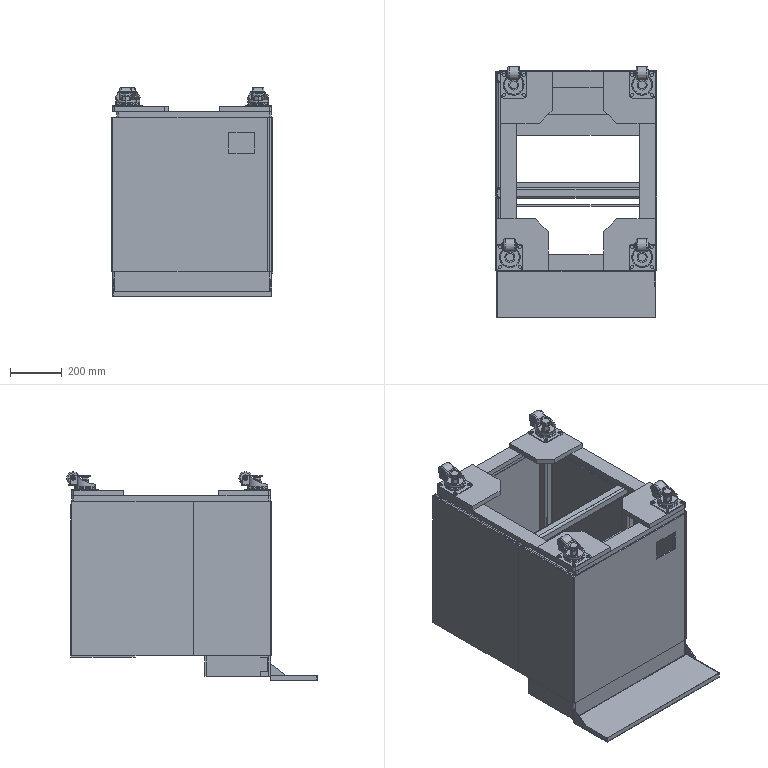Assembly | SolidWorks | mm | 31 component files | 63 solids | 1320 faces | box 625 x 971.67 x 809 mm | volume 27248260 mm3 | plane 703 | cylinder 457 | cone 96 | torus 64 | commonest cylinder face diameters 16 x106 8 x80 11 x48 13 x32 20 x20 80 x16 24 x16 25 x16
Bill of materials:
CMAS50_Fadjuster | 4 | 45 | Headed pin or bolt-like part: a thin, wide, round head with a slightly tapered underside, a hexagonal neck section under the head, and a long plain cylindrical shank with a chamfered end.
CMAS50_Fbearing | 4 | 45 | Stepped cylinder: a large main cylinder with a shorter, smaller coaxial cylindrical spigot sticking out of each end.
CMAS50_Fbody | 4 | 45 | Bracket with a circular base and a central hexagonal boss with a through-hole. A curved wall rises from the base to two parallel upright ears, each with a round boss or pivot feature.
CMAS50_Fswivel | 4 | 45 | Square flange plate with rounded corners, four slotted holes at the corners, and a raised circular disc with a central round through-hole.
CMAS50_Fwheel | 4 | 45 | Cylindrical sleeve or bushing with a central through-bore and rounded outer edges.
CoverPlate1 | 2 |  | Thin flat rectangular plate, about twice as long as it is wide, with no visible features.
CoverPlate2 | 2 |  | Thin flat rectangular plate, slightly taller than it is wide, with no visible features.
CoverPlate3 | 1 |  | Thin flat square plate with one small rectangular through-cutout near one corner.
CoverPlate4 | 1 |  | Thin flat square plate with no visible features.
CoverPlate5 | 1 |  | Thin flat rectangular strip or panel, about 3.5 times as long as it is wide, with no visible features.
CoverPlate6 | 2 |  | Long, narrow, thin flat strip or bar with no visible features.
ItemTray | 1 |  | Rectangular plate with a thin triangular flange or gusset standing up at each short end, placed toward one long edge.
STRack | 1 |  | Open rectangular box frame made of square/rectangular bar members: four vertical corner posts, top and bottom perimeter rails, and an intermediate vertical post with a cross rail that splits the frame into two bays. Square corner plates with chamfered inner corners and a single small hole each sit on the top corners. A flat vertical panel with a few small holes fills part of one side, and a solid rectangular base block sits under one corner.
Mates:
1. coincident | STRack-1 face at (-277, 602, 620) dir (0, 0, 1) | CMAS50_F-4/CMAS50_Fswivel-1 face at (-273, 520, 620) dir (0, 0, -1)
2. coincident | STRack-1 face at (-285, 602, 620) dir (-1, 0, 0) | CMAS50_F-4/CMAS50_Fswivel-1 face at (-285, 520, 623.2) dir (-1, 0, 0)
3. coincident | STRack-1 face at (-277, 610, 620) dir (0, 1, 0) | CMAS50_F-4/CMAS50_Fswivel-1 face at (-273, 610, 623.2) dir (0, 1, 0)
4. coincident | STRack-1 face at (307, 602, 620) dir (0, 0, 1) | CMAS50_F-2/CMAS50_Fswivel-1 face at (225, 520, 620) dir (0, 0, -1)
5. coincident | STRack-1 face at (315, 602, 620) dir (1, 0, 0) | CMAS50_F-2/CMAS50_Fswivel-1 face at (315, 598, 623.2) dir (1, 0, 0)
6. coincident | STRack-1 face at (307, 610, 620) dir (0, 1, 0) | CMAS50_F-2/CMAS50_Fswivel-1 face at (225, 610, 623.2) dir (0, 1, 0)
7. coincident | STRack-1 face at (-292, -152, 620) dir (0, 0, 1) | CMAS50_F-3/CMAS50_Fswivel-1 face at (-288, -148, 620) dir (0, 0, -1)
8. coincident | STRack-1 face at (-300, -152, 620) dir (-1, 0, 0) | CMAS50_F-3/CMAS50_Fswivel-1 face at (-300, -148, 623.2) dir (-1, 0, 0)
9. coincident | STRack-1 face at (-292, -160, 620) dir (0, -1, 0) | CMAS50_F-3/CMAS50_Fswivel-1 face at (-210, -160, 623.2) dir (0, -1, 0)
10. coincident | STRack-1 face at (-300, 140, 12) dir (-1, 0, 0) | CoverPlate1-1 face at (-300, -10, 280) dir (1, 0, 0)
11. coincident | STRack-1 edge at (-285, 602, 580) dir (0, -1, 0) | CoverPlate1-1 face at (-300, -160, 580) dir (0, 0, 1)
12. coincident | STRack-1 face at (-292, -160, 560) dir (0, -1, 0) | CoverPlate1-1 face at (-300, -160, 580) dir (0, -1, 0)
13. coincident | STRack-1 face at (315, 152, 560) dir (1, 0, 0) | CoverPlate1-2 face at (315, -10, 280) dir (-1, 0, 0)
14. coincident | STRack-1 face at (0, 0, 580) dir (0, 0, -1) | CoverPlate1-2 face at (320, -160, 580) dir (0, 0, 1)
15. coincident | STRack-1 face at (283, -160, 560) dir (0, -1, 0) | CoverPlate1-2 face at (320, -160, 580) dir (0, -1, 0)
16. coincident | STRack-1 face at (315, 590, 548) dir (1, 0, 0) | CoverPlate2-1 face at (315, 375, 280) dir (-1, 0, 0)
17. coincident | CoverPlate1-2 face at (320, 140, 580) dir (0, 1, 0) | CoverPlate2-1 face at (320, 140, 580) dir (0, -1, 0)
18. coincident | STRack-1 face at (283, 180, -20) dir (0, 0, -1) | CoverPlate2-1 face at (320, 140, -20) dir (0, 0, -1)
19. coincident | STRack-1 face at (-300, 180, -12) dir (-1, 0, 0) | CoverPlate2-2 face at (-300, 375, 280) dir (1, 0, 0)
20. coincident | CoverPlate1-1 face at (-300, 140, 580) dir (0, 1, 0) | CoverPlate2-2 face at (-300, 140, 580) dir (0, -1, 0)
21. coincident | STRack-1 face at (0, 0, 580) dir (0, 0, -1) | CoverPlate2-2 face at (-300, 140, 580) dir (0, 0, 1)
22. coincident | STRack-1 face at (-280, -160, 548) dir (0, -1, 0) | CoverPlate3-1 face at (0, -160, 280) dir (0, 1, 0)
23. coincident | STRack-1 face at (0, 0, 580) dir (0, 0, -1) | CoverPlate3-1 face at (-300, -160, 580) dir (0, 0, 1)
24. coincident | CoverPlate1-1 face at (-300, -10, 280) dir (1, 0, 0) | CoverPlate3-1 face at (-300, -160, -20) dir (-1, 0, 0)
25. coincident | STRack-1 face at (295, 610, 548) dir (0, 1, 0) | CoverPlate4-1 face at (15, 610, 272.5) dir (0, -1, 0)
26. tangent | STRack-1 face at (295, 578, -12) dir (-1, 0, 0) r 8 | CoverPlate4-1 face at (-285, 615, -20) dir (0, 0, -1)
27. coincident | CoverPlate2-1 face at (315, 375, 280) dir (-1, 0, 0) | CoverPlate4-1 face at (315, 615, -20) dir (1, 0, 0)
28. coincident | STRack-1 face at (-292, 180, -20) dir (0, 0, -1) | CoverPlate5-1 face at (15, 530, -20) dir (0, 0, 1)
29. coincident | CoverPlate2-1 face at (320, 375, 280) dir (1, 0, 0) | CoverPlate5-1 face at (320, 615, -20) dir (1, 0, 0)
30. coincident | CoverPlate4-1 face at (15, 615, 272.5) dir (0, 1, 0) | CoverPlate5-1 face at (-290, 615, -20) dir (0, 1, 0)
31. coincident | STRack-1 face at (0, 90, 0) dir (0, 1, 0) | CoverPlate6-1 face at (15, 90, -60) dir (0, -1, 0)
32. coincident | STRack-1 face at (283, -140, -20) dir (0, 0, -1) | CoverPlate6-1 face at (-285, 95, -20) dir (0, 0, 1)
33. coincident | STRack-1 face at (315, 90, -100) dir (1, 0, 0) | CoverPlate6-1 face at (315, 95, -100) dir (1, 0, 0)
34. coincident | STRack-1 face at (-292, 180, -20) dir (0, 0, -1) | CoverPlate6-2 face at (15, 405, -20) dir (0, 0, 1)
35. coincident | CoverPlate5-1 face at (-290, 445, -20) dir (0, -1, 0) | CoverPlate6-2 face at (-285, 445, -25) dir (0, 1, 0)
36. width | CoverPlate5-1 face at (320, 615, -20) dir (1, 0, 0) | CoverPlate5-1 face at (-290, 615, -20) dir (-1, 0, 0) | CoverPlate6-2 face at (315, 365, -25) dir (1, 0, 0) | CoverPlate6-2 face at (-285, 365, -25) dir (-1, 0, 0)
37. coincident | CMAS50_Fswivel-1 plane at (264, -109, 632.8) dir (0, 0, -1) | CMAS50_Fbody-1 plane at (264, -109, 632.8) dir (0, 0, -1)
38. coincident | CMAS50_Fswivel-1 axis at (264, -109, 570) dir (0, 0, 1) | CMAS50_Fbody-1 axis at (264, -109, 570) dir (0, 0, 1)
39. coincident | CMAS50_Fbody-1 plane at (264, -109, 620) dir (1, 0.009642, 0) | CMAS50_Fbearing-1 plane at (263.556, -63.002, 669) dir (-1, -0.009642, 0)
40. coincident | CMAS50_Fbody-1 axis at (344.453, -62.222, 669) dir (-1, -0.009642, 0) | CMAS50_Fbearing-1 axis at (182.66, -63.782, 669) dir (1, 0.009642, 0)
41. coincident | CMAS50_Fbody-1 axis at (264, -109, 570) dir (0, 0, 1) | CMAS50_Fadjuster-1 axis at (264, -109, 570) dir (0, 0, 1)
42. distance | CMAS50_Fwheel-1 plane at (263.556, -63.002, 669) dir (1, 0.009642, 0) | CMAS50_Fbearing-1 plane at (263.556, -63.002, 669) dir (-1, -0.009642, 0)
43. coincident | CMAS50_Fbearing-1 axis at (182.66, -63.782, 669) dir (1, 0.009642, 0) | CMAS50_Fwheel-1 axis at (344.453, -62.222, 669) dir (-1, -0.009642, 0)
44. coincident | CMAS50_Fbearing-1 axis at (182.66, -63.782, 669) dir (1, 0.009642, 0) | CMAS50_Fwheel-1 axis at (344.453, -62.222, 669) dir (-1, -0.009642, 0)
45. coincident | CMAS50_Fbearing-1 axis at (182.66, -63.782, 669) dir (1, 0.009642, 0) | CMAS50_Fwheel-1 axis at (344.453, -62.222, 669) dir (-1, -0.009642, 0)
46. angle | CMAS50_Fwheel-1 plane at (263.556, -63.002, 669) dir (-0.00848, 0.8794, -0.476) | CMAS50_Fbearing-1 plane at (263.556, -63.002, 669) dir (-0.00848, 0.8794, -0.476)
47. coincident | STRack-1 face at (307, -152, 620) dir (0, 0, 1) | CMAS50_Fswivel-1 face at (225, -148, 620) dir (0, 0, -1)
48. coincident | STRack-1 face at (315, -152, 620) dir (1, 0, 0) | CMAS50_Fswivel-1 face at (315, -70, 623.2) dir (1, 0, 0)
49. coincident | STRack-1 face at (307, -160, 620) dir (0, -1, 0) | CMAS50_Fswivel-1 face at (303, -160, 623.2) dir (0, -1, 0)
50. coincident | CMAS50_Fswivel-1 plane at (0, -12.8, 0) dir (0, 1, 0) | CMAS50_Fbody-1 plane at (0, -12.8, 0) dir (0, 1, 0)
51. coincident | CMAS50_Fswivel-1 axis at (0, 50, 0) dir (0, -1, 0) | CMAS50_Fbody-1 axis at (0, 50, 0) dir (0, -1, 0)
52. coincident | CMAS50_Fbody-1 plane at (0, 0, 0) dir (1, 0, 0.009642) | CMAS50_Fbearing-1 plane at (-0.4435, -49, 45.998) dir (-1, 0, -0.009642)
53. coincident | CMAS50_Fbody-1 axis at (80.453, -49, 46.778) dir (-1, 0, -0.009642) | CMAS50_Fbearing-1 axis at (-81.34, -49, 45.218) dir (1, 0, 0.009642)
54. distance | CMAS50_Fwheel-1 plane at (-0.4435, -49, 45.998) dir (1, 0, 0.009642) | CMAS50_Fbearing-1 plane at (-0.4435, -49, 45.998) dir (-1, 0, -0.009642)
55. coincident | CMAS50_Fbearing-1 axis at (-81.34, -49, 45.218) dir (1, 0, 0.009642) | CMAS50_Fwheel-1 axis at (80.453, -49, 46.778) dir (-1, 0, -0.009642)
56. coincident | CMAS50_Fbearing-1 axis at (-81.34, -49, 45.218) dir (1, 0, 0.009642) | CMAS50_Fwheel-1 axis at (80.453, -49, 46.778) dir (-1, 0, -0.009642)
57. coincident | CMAS50_Fbearing-1 axis at (-81.34, -49, 45.218) dir (1, 0, 0.009642) | CMAS50_Fwheel-1 axis at (80.453, -49, 46.778) dir (-1, 0, -0.009642)
58. angle | CMAS50_Fwheel-1 plane at (-0.4435, -49, 45.998) dir (-0.00848, 0.476, 0.8794) | CMAS50_Fbearing-1 plane at (-0.4435, -49, 45.998) dir (-0.00848, 0.476, 0.8794)
59. coincident | CMAS50_Fbody-1 axis at (0, 50, 0) dir (0, -1, 0) | CMAS50_Fadjuster-1 axis at (0, 50, 0) dir (0, -1, 0)